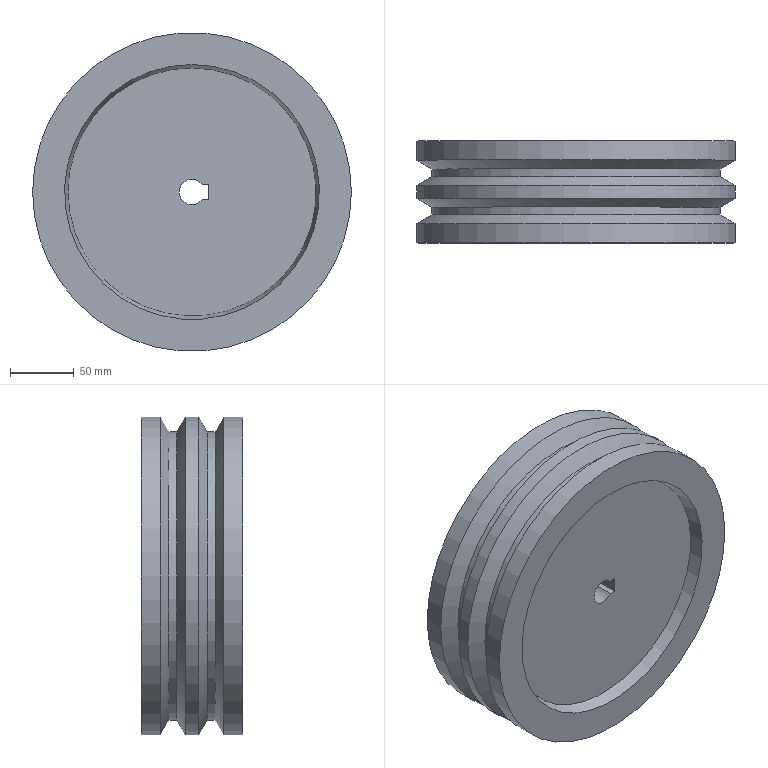Component | NX | DRIVEN_WHEEL | 1 solid | 19 faces | volume 3057229 mm3 | plane 7 | cylinder 6 | cone 6 | commonest cylinder face diameters 250 x3 226 x2 20 x1